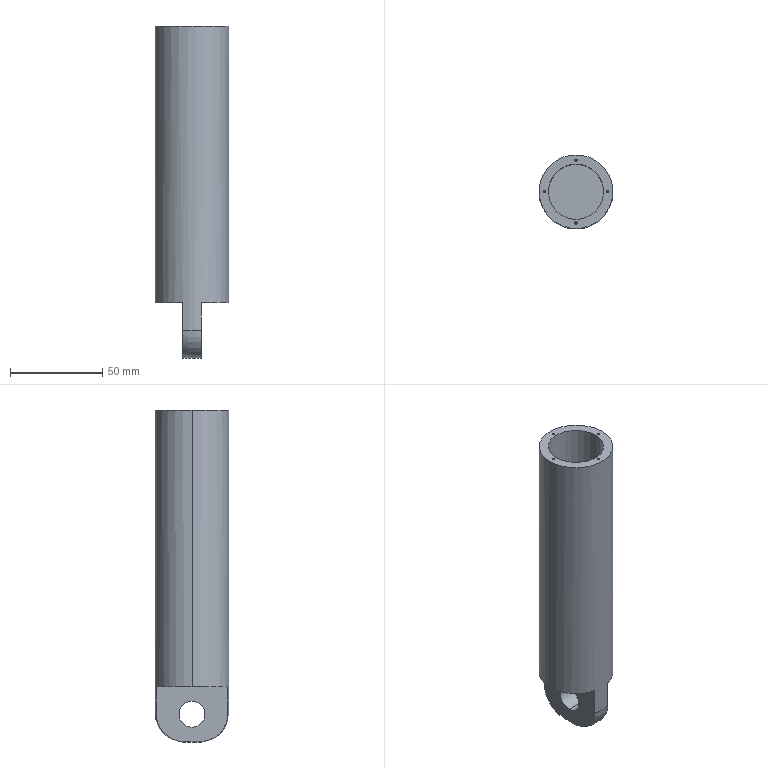Component | SolidWorks | CylinderBody-1 | 1 solid | 31 faces | box 40 x 40 x 180 mm | volume 98862 mm3 | cylinder 14 | cone 8 | plane 7 | torus 2 | commonest cylinder face diameters 1.25 x8 30 x2 14 x2 40 x2
STEP:
#1=CARTESIAN_POINT('',(0.8858,-0.06482,8.959));
#2=VERTEX_POINT('',#1);
#3=CARTESIAN_POINT('',(0.935,-0.06482,8.959));
#4=VERTEX_POINT('',#3);
#5=CARTESIAN_POINT('',(0.9104,-0.06482,8.959));
#6=DIRECTION('',(0.,0.,1.));
#7=DIRECTION('',(1.,0.,0.));
#8=AXIS2_PLACEMENT_3D('',#5,#6,#7);
#9=CIRCLE('',#8,0.02461);
#10=EDGE_CURVE('',#2,#4,#9,.T.);
#11=ORIENTED_EDGE('',*,*,#10,.F.);
#12=CARTESIAN_POINT('',(0.8858,-0.06482,9.154));
#13=VERTEX_POINT('',#12);
#14=CARTESIAN_POINT('',(0.8858,-0.06482,9.154));
#15=DIRECTION('',(0.,0.,1.));
#16=VECTOR('',#15,39.37);
#17=LINE('',#14,#16);
#18=EDGE_CURVE('',#2,#13,#17,.T.);
#19=ORIENTED_EDGE('',*,*,#18,.T.);
#20=CARTESIAN_POINT('',(0.935,-0.06482,9.154));
#21=VERTEX_POINT('',#20);
#22=CARTESIAN_POINT('',(0.9104,-0.06482,9.154));
#23=DIRECTION('',(0.,0.,1.));
#24=DIRECTION('',(1.,0.,0.));
#25=AXIS2_PLACEMENT_3D('',#22,#23,#24);
#26=CIRCLE('',#25,0.02461);
#27=EDGE_CURVE('',#13,#21,#26,.T.);
#28=ORIENTED_EDGE('',*,*,#27,.T.);
#29=CARTESIAN_POINT('',(0.935,-0.06482,9.154));
#30=DIRECTION('',(0.,0.,1.));
#31=VECTOR('',#30,39.37);
#32=LINE('',#29,#31);
#33=EDGE_CURVE('',#4,#21,#32,.T.);
#34=ORIENTED_EDGE('',*,*,#33,.F.);
#35=EDGE_LOOP('',(#11,#19,#28,#34));
#36=FACE_OUTER_BOUND('',#35,.T.);
#37=CARTESIAN_POINT('',(0.9104,-0.06482,9.154));
#38=DIRECTION('',(0.,0.,1.));
#39=DIRECTION('',(1.,0.,0.));
#40=AXIS2_PLACEMENT_3D('',#37,#38,#39);
#41=CYLINDRICAL_SURFACE('',#40,0.02461);
#42=ADVANCED_FACE('',(#36),#41,.F.);
#43=CARTESIAN_POINT('',(0.9104,-0.06482,8.944));
#44=VERTEX_POINT('',#43);
#45=CARTESIAN_POINT('',(0.935,-0.06482,8.959));
#46=DIRECTION('',(0.8572,0.,0.515));
#47=VECTOR('',#46,39.37);
#48=LINE('',#45,#47);
#49=EDGE_CURVE('',#44,#4,#48,.T.);
#50=ORIENTED_EDGE('',*,*,#49,.F.);
#51=CARTESIAN_POINT('',(0.8858,-0.06482,8.959));
#52=DIRECTION('',(-0.8572,0.,0.515));
#53=VECTOR('',#52,39.37);
#54=LINE('',#51,#53);
#55=EDGE_CURVE('',#44,#2,#54,.T.);
#56=ORIENTED_EDGE('',*,*,#55,.T.);
#57=ORIENTED_EDGE('',*,*,#10,.T.);
#58=EDGE_LOOP('',(#50,#56,#57));
#59=FACE_OUTER_BOUND('',#58,.T.);
#60=CARTESIAN_POINT('',(0.9104,-0.06482,8.959));
#61=DIRECTION('',(0.,0.,1.));
#62=DIRECTION('',(1.,0.,0.));
#63=AXIS2_PLACEMENT_3D('',#60,#61,#62);
#64=CONICAL_SURFACE('',#63,0.02461,1.03);
#65=ADVANCED_FACE('',(#59),#64,.F.);
#66=CARTESIAN_POINT('',(0.2165,-0.7341,8.959));
#67=VERTEX_POINT('',#66);
#68=CARTESIAN_POINT('',(0.2657,-0.7341,8.959));
#69=VERTEX_POINT('',#68);
#70=CARTESIAN_POINT('',(0.2411,-0.7341,8.959));
#71=DIRECTION('',(0.,0.,1.));
#72=DIRECTION('',(1.,0.,0.));
#73=AXIS2_PLACEMENT_3D('',#70,#71,#72);
#74=CIRCLE('',#73,0.02461);
#75=EDGE_CURVE('',#67,#69,#74,.T.);
#76=ORIENTED_EDGE('',*,*,#75,.F.);
#77=CARTESIAN_POINT('',(0.2165,-0.7341,9.154));
#78=VERTEX_POINT('',#77);
#79=CARTESIAN_POINT('',(0.2165,-0.7341,9.154));
#80=DIRECTION('',(0.,0.,1.));
#81=VECTOR('',#80,39.37);
#82=LINE('',#79,#81);
#83=EDGE_CURVE('',#67,#78,#82,.T.);
#84=ORIENTED_EDGE('',*,*,#83,.T.);
#85=CARTESIAN_POINT('',(0.2657,-0.7341,9.154));
#86=VERTEX_POINT('',#85);
#87=CARTESIAN_POINT('',(0.2411,-0.7341,9.154));
#88=DIRECTION('',(0.,0.,1.));
#89=DIRECTION('',(1.,0.,0.));
#90=AXIS2_PLACEMENT_3D('',#87,#88,#89);
#91=CIRCLE('',#90,0.02461);
#92=EDGE_CURVE('',#78,#86,#91,.T.);
#93=ORIENTED_EDGE('',*,*,#92,.T.);
#94=CARTESIAN_POINT('',(0.2657,-0.7341,9.154));
#95=DIRECTION('',(0.,0.,1.));
#96=VECTOR('',#95,39.37);
#97=LINE('',#94,#96);
#98=EDGE_CURVE('',#69,#86,#97,.T.);
#99=ORIENTED_EDGE('',*,*,#98,.F.);
#100=EDGE_LOOP('',(#76,#84,#93,#99));
#101=FACE_OUTER_BOUND('',#100,.T.);
#102=CARTESIAN_POINT('',(0.2411,-0.7341,9.154));
#103=DIRECTION('',(0.,0.,1.));
#104=DIRECTION('',(1.,0.,0.));
#105=AXIS2_PLACEMENT_3D('',#102,#103,#104);
#106=CYLINDRICAL_SURFACE('',#105,0.02461);
#107=ADVANCED_FACE('',(#101),#106,.F.);
#108=CARTESIAN_POINT('',(0.2411,-0.7341,8.944));
#109=VERTEX_POINT('',#108);
#110=CARTESIAN_POINT('',(0.2657,-0.7341,8.959));
#111=DIRECTION('',(0.8572,0.,0.515));
#112=VECTOR('',#111,39.37);
#113=LINE('',#110,#112);
#114=EDGE_CURVE('',#109,#69,#113,.T.);
#115=ORIENTED_EDGE('',*,*,#114,.F.);
#116=CARTESIAN_POINT('',(0.2165,-0.7341,8.959));
#117=DIRECTION('',(-0.8572,0.,0.515));
#118=VECTOR('',#117,39.37);
#119=LINE('',#116,#118);
#120=EDGE_CURVE('',#109,#67,#119,.T.);
#121=ORIENTED_EDGE('',*,*,#120,.T.);
#122=ORIENTED_EDGE('',*,*,#75,.T.);
#123=EDGE_LOOP('',(#115,#121,#122));
#124=FACE_OUTER_BOUND('',#123,.T.);
#125=CARTESIAN_POINT('',(0.2411,-0.7341,8.959));
#126=DIRECTION('',(0.,0.,1.));
#127=DIRECTION('',(1.,0.,0.));
#128=AXIS2_PLACEMENT_3D('',#125,#126,#127);
#129=CONICAL_SURFACE('',#128,0.02461,1.03);
#130=ADVANCED_FACE('',(#124),#129,.F.);
#131=CARTESIAN_POINT('',(-0.4528,-0.06482,8.959));
#132=VERTEX_POINT('',#131);
#133=CARTESIAN_POINT('',(-0.4035,-0.06482,8.959));
#134=VERTEX_POINT('',#133);
#135=CARTESIAN_POINT('',(-0.4282,-0.06482,8.959));
#136=DIRECTION('',(0.,0.,1.));
#137=DIRECTION('',(1.,0.,0.));
#138=AXIS2_PLACEMENT_3D('',#135,#136,#137);
#139=CIRCLE('',#138,0.02461);
#140=EDGE_CURVE('',#132,#134,#139,.T.);
#141=ORIENTED_EDGE('',*,*,#140,.F.);
#142=CARTESIAN_POINT('',(-0.4528,-0.06482,9.154));
#143=VERTEX_POINT('',#142);
#144=CARTESIAN_POINT('',(-0.4528,-0.06482,9.154));
#145=DIRECTION('',(0.,0.,1.));
#146=VECTOR('',#145,39.37);
#147=LINE('',#144,#146);
#148=EDGE_CURVE('',#132,#143,#147,.T.);
#149=ORIENTED_EDGE('',*,*,#148,.T.);
#150=CARTESIAN_POINT('',(-0.4035,-0.06482,9.154));
#151=VERTEX_POINT('',#150);
#152=CARTESIAN_POINT('',(-0.4282,-0.06482,9.154));
#153=DIRECTION('',(0.,0.,1.));
#154=DIRECTION('',(1.,0.,0.));
#155=AXIS2_PLACEMENT_3D('',#152,#153,#154);
#156=CIRCLE('',#155,0.02461);
#157=EDGE_CURVE('',#143,#151,#156,.T.);
#158=ORIENTED_EDGE('',*,*,#157,.T.);
#159=CARTESIAN_POINT('',(-0.4035,-0.06482,9.154));
#160=DIRECTION('',(0.,0.,1.));
#161=VECTOR('',#160,39.37);
#162=LINE('',#159,#161);
#163=EDGE_CURVE('',#134,#151,#162,.T.);
#164=ORIENTED_EDGE('',*,*,#163,.F.);
#165=EDGE_LOOP('',(#141,#149,#158,#164));
#166=FACE_OUTER_BOUND('',#165,.T.);
#167=CARTESIAN_POINT('',(-0.4282,-0.06482,9.154));
#168=DIRECTION('',(0.,0.,1.));
#169=DIRECTION('',(1.,0.,0.));
#170=AXIS2_PLACEMENT_3D('',#167,#168,#169);
#171=CYLINDRICAL_SURFACE('',#170,0.02461);
#172=ADVANCED_FACE('',(#166),#171,.F.);
#173=CARTESIAN_POINT('',(-0.4282,-0.06482,8.944));
#174=VERTEX_POINT('',#173);
#175=CARTESIAN_POINT('',(-0.4035,-0.06482,8.959));
#176=DIRECTION('',(0.8572,0.,0.515));
#177=VECTOR('',#176,39.37);
#178=LINE('',#175,#177);
#179=EDGE_CURVE('',#174,#134,#178,.T.);
#180=ORIENTED_EDGE('',*,*,#179,.F.);
#181=CARTESIAN_POINT('',(-0.4528,-0.06482,8.959));
#182=DIRECTION('',(-0.8572,0.,0.515));
#183=VECTOR('',#182,39.37);
#184=LINE('',#181,#183);
#185=EDGE_CURVE('',#174,#132,#184,.T.);
#186=ORIENTED_EDGE('',*,*,#185,.T.);
#187=ORIENTED_EDGE('',*,*,#140,.T.);
#188=EDGE_LOOP('',(#180,#186,#187));
#189=FACE_OUTER_BOUND('',#188,.T.);
#190=CARTESIAN_POINT('',(-0.4282,-0.06482,8.959));
#191=DIRECTION('',(0.,0.,1.));
#192=DIRECTION('',(1.,0.,0.));
#193=AXIS2_PLACEMENT_3D('',#190,#191,#192);
#194=CONICAL_SURFACE('',#193,0.02461,1.03);
#195=ADVANCED_FACE('',(#189),#194,.F.);
#196=CARTESIAN_POINT('',(0.2165,0.6045,8.959));
#197=VERTEX_POINT('',#196);
#198=CARTESIAN_POINT('',(0.2657,0.6045,8.959));
#199=VERTEX_POINT('',#198);
#200=CARTESIAN_POINT('',(0.2411,0.6045,8.959));
#201=DIRECTION('',(0.,0.,1.));
#202=DIRECTION('',(1.,0.,0.));
#203=AXIS2_PLACEMENT_3D('',#200,#201,#202);
#204=CIRCLE('',#203,0.02461);
#205=EDGE_CURVE('',#197,#199,#204,.T.);
#206=ORIENTED_EDGE('',*,*,#205,.F.);
#207=CARTESIAN_POINT('',(0.2165,0.6045,9.154));
#208=VERTEX_POINT('',#207);
#209=CARTESIAN_POINT('',(0.2165,0.6045,9.154));
#210=DIRECTION('',(0.,0.,1.));
#211=VECTOR('',#210,39.37);
#212=LINE('',#209,#211);
#213=EDGE_CURVE('',#197,#208,#212,.T.);
#214=ORIENTED_EDGE('',*,*,#213,.T.);
#215=CARTESIAN_POINT('',(0.2657,0.6045,9.154));
#216=VERTEX_POINT('',#215);
#217=CARTESIAN_POINT('',(0.2411,0.6045,9.154));
#218=DIRECTION('',(0.,0.,1.));
#219=DIRECTION('',(1.,0.,0.));
#220=AXIS2_PLACEMENT_3D('',#217,#218,#219);
#221=CIRCLE('',#220,0.02461);
#222=EDGE_CURVE('',#208,#216,#221,.T.);
#223=ORIENTED_EDGE('',*,*,#222,.T.);
#224=CARTESIAN_POINT('',(0.2657,0.6045,9.154));
#225=DIRECTION('',(0.,0.,1.));
#226=VECTOR('',#225,39.37);
#227=LINE('',#224,#226);
#228=EDGE_CURVE('',#199,#216,#227,.T.);
#229=ORIENTED_EDGE('',*,*,#228,.F.);
#230=EDGE_LOOP('',(#206,#214,#223,#229));
#231=FACE_OUTER_BOUND('',#230,.T.);
#232=CARTESIAN_POINT('',(0.2411,0.6045,9.154));
#233=DIRECTION('',(0.,0.,1.));
#234=DIRECTION('',(1.,0.,0.));
#235=AXIS2_PLACEMENT_3D('',#232,#233,#234);
#236=CYLINDRICAL_SURFACE('',#235,0.02461);
#237=ADVANCED_FACE('',(#231),#236,.F.);
#238=CARTESIAN_POINT('',(0.2411,0.6045,8.944));
#239=VERTEX_POINT('',#238);
#240=CARTESIAN_POINT('',(0.2657,0.6045,8.959));
#241=DIRECTION('',(0.8572,0.,0.515));
#242=VECTOR('',#241,39.37);
#243=LINE('',#240,#242);
#244=EDGE_CURVE('',#239,#199,#243,.T.);
#245=ORIENTED_EDGE('',*,*,#244,.F.);
#246=CARTESIAN_POINT('',(0.2165,0.6045,8.959));
#247=DIRECTION('',(-0.8572,0.,0.515));
#248=VECTOR('',#247,39.37);
#249=LINE('',#246,#248);
#250=EDGE_CURVE('',#239,#197,#249,.T.);
#251=ORIENTED_EDGE('',*,*,#250,.T.);
#252=ORIENTED_EDGE('',*,*,#205,.T.);
#253=EDGE_LOOP('',(#245,#251,#252));
#254=FACE_OUTER_BOUND('',#253,.T.);
#255=CARTESIAN_POINT('',(0.2411,0.6045,8.959));
#256=DIRECTION('',(0.,0.,1.));
#257=DIRECTION('',(1.,0.,0.));
#258=AXIS2_PLACEMENT_3D('',#255,#256,#257);
#259=CONICAL_SURFACE('',#258,0.02461,1.03);
#260=ADVANCED_FACE('',(#254),#259,.F.);
#261=CARTESIAN_POINT('',(-0.3494,-0.06482,3.642));
#262=VERTEX_POINT('',#261);
#263=CARTESIAN_POINT('',(0.8317,-0.06482,3.642));
#264=VERTEX_POINT('',#263);
#265=CARTESIAN_POINT('',(0.2411,-0.06482,3.642));
#266=DIRECTION('',(0.,0.,1.));
#267=DIRECTION('',(1.,0.,0.));
#268=AXIS2_PLACEMENT_3D('',#265,#266,#267);
#269=CIRCLE('',#268,0.5906);
#270=EDGE_CURVE('',#262,#264,#269,.T.);
#271=ORIENTED_EDGE('',*,*,#270,.F.);
#272=CARTESIAN_POINT('',(-0.3494,-0.06482,9.154));
#273=VERTEX_POINT('',#272);
#274=CARTESIAN_POINT('',(-0.3494,-0.06482,3.642));
#275=DIRECTION('',(0.,0.,1.));
#276=VECTOR('',#275,39.37);
#277=LINE('',#274,#276);
#278=EDGE_CURVE('',#262,#273,#277,.T.);
#279=ORIENTED_EDGE('',*,*,#278,.T.);
#280=CARTESIAN_POINT('',(0.8317,-0.06482,9.154));
#281=VERTEX_POINT('',#280);
#282=CARTESIAN_POINT('',(0.2411,-0.06482,9.154));
#283=DIRECTION('',(0.,0.,1.));
#284=DIRECTION('',(1.,0.,0.));
#285=AXIS2_PLACEMENT_3D('',#282,#283,#284);
#286=CIRCLE('',#285,0.5906);
#287=EDGE_CURVE('',#273,#281,#286,.T.);
#288=ORIENTED_EDGE('',*,*,#287,.T.);
#289=CARTESIAN_POINT('',(0.8317,-0.06482,3.642));
#290=DIRECTION('',(0.,0.,1.));
#291=VECTOR('',#290,39.37);
#292=LINE('',#289,#291);
#293=EDGE_CURVE('',#264,#281,#292,.T.);
#294=ORIENTED_EDGE('',*,*,#293,.F.);
#295=EDGE_LOOP('',(#271,#279,#288,#294));
#296=FACE_OUTER_BOUND('',#295,.T.);
#297=CARTESIAN_POINT('',(0.2411,-0.06482,3.642));
#298=DIRECTION('',(0.,0.,1.));
#299=DIRECTION('',(1.,0.,0.));
#300=AXIS2_PLACEMENT_3D('',#297,#298,#299);
#301=CYLINDRICAL_SURFACE('',#300,0.5906);
#302=ADVANCED_FACE('',(#296),#301,.F.);
#303=CARTESIAN_POINT('',(0.438,-0.06482,2.382));
#304=VERTEX_POINT('',#303);
#305=CARTESIAN_POINT('',(0.438,-0.06482,2.933));
#306=VERTEX_POINT('',#305);
#307=CARTESIAN_POINT('',(0.438,-0.06482,2.657));
#308=DIRECTION('',(-1.,0.,0.));
#309=DIRECTION('',(0.,0.,1.));
#310=AXIS2_PLACEMENT_3D('',#307,#308,#309);
#311=CIRCLE('',#310,0.2756);
#312=EDGE_CURVE('',#304,#306,#311,.T.);
#313=ORIENTED_EDGE('',*,*,#312,.F.);
#314=CARTESIAN_POINT('',(0.04429,-0.06482,2.382));
#315=VERTEX_POINT('',#314);
#316=CARTESIAN_POINT('',(1.029,-0.06482,2.382));
#317=DIRECTION('',(-1.,0.,0.));
#318=VECTOR('',#317,39.37);
#319=LINE('',#316,#318);
#320=EDGE_CURVE('',#304,#315,#319,.T.);
#321=ORIENTED_EDGE('',*,*,#320,.T.);
#322=CARTESIAN_POINT('',(0.04429,-0.06482,2.933));
#323=VERTEX_POINT('',#322);
#324=CARTESIAN_POINT('',(0.04429,-0.06482,2.657));
#325=DIRECTION('',(-1.,0.,0.));
#326=DIRECTION('',(0.,0.,1.));
#327=AXIS2_PLACEMENT_3D('',#324,#325,#326);
#328=CIRCLE('',#327,0.2756);
#329=EDGE_CURVE('',#315,#323,#328,.T.);
#330=ORIENTED_EDGE('',*,*,#329,.T.);
#331=CARTESIAN_POINT('',(1.029,-0.06482,2.933));
#332=DIRECTION('',(-1.,0.,0.));
#333=VECTOR('',#332,39.37);
#334=LINE('',#331,#333);
#335=EDGE_CURVE('',#306,#323,#334,.T.);
#336=ORIENTED_EDGE('',*,*,#335,.F.);
#337=EDGE_LOOP('',(#313,#321,#330,#336));
#338=FACE_OUTER_BOUND('',#337,.T.);
#339=CARTESIAN_POINT('',(1.029,-0.06482,2.657));
#340=DIRECTION('',(-1.,0.,0.));
#341=DIRECTION('',(0.,0.,1.));
#342=AXIS2_PLACEMENT_3D('',#339,#340,#341);
#343=CYLINDRICAL_SURFACE('',#342,0.2756);
#344=ADVANCED_FACE('',(#338),#343,.F.);
#345=CARTESIAN_POINT('',(1.029,-0.06482,9.154));
#346=VERTEX_POINT('',#345);
#347=CARTESIAN_POINT('',(-0.5463,-0.06482,9.154));
#348=VERTEX_POINT('',#347);
#349=CARTESIAN_POINT('',(0.2411,-0.06482,9.154));
#350=DIRECTION('',(0.,0.,1.));
#351=DIRECTION('',(1.,0.,0.));
#352=AXIS2_PLACEMENT_3D('',#349,#350,#351);
#353=CIRCLE('',#352,0.7874);
#354=EDGE_CURVE('',#346,#348,#353,.T.);
#355=ORIENTED_EDGE('',*,*,#354,.F.);
#356=CARTESIAN_POINT('',(1.029,-0.06482,3.248));
#357=VERTEX_POINT('',#356);
#358=CARTESIAN_POINT('',(1.029,-0.06482,9.154));
#359=DIRECTION('',(0.,0.,-1.));
#360=VECTOR('',#359,39.37);
#361=LINE('',#358,#360);
#362=EDGE_CURVE('',#346,#357,#361,.T.);
#363=ORIENTED_EDGE('',*,*,#362,.T.);
#364=CARTESIAN_POINT('',(0.438,0.6976,3.248));
#365=VERTEX_POINT('',#364);
#366=CARTESIAN_POINT('',(0.2411,-0.06482,3.248));
#367=DIRECTION('',(0.,0.,1.));
#368=DIRECTION('',(1.,0.,0.));
#369=AXIS2_PLACEMENT_3D('',#366,#367,#368);
#370=CIRCLE('',#369,0.7874);
#371=EDGE_CURVE('',#357,#365,#370,.T.);
#372=ORIENTED_EDGE('',*,*,#371,.T.);
#373=CARTESIAN_POINT('',(0.438,0.6976,2.657));
#374=VERTEX_POINT('',#373);
#375=CARTESIAN_POINT('',(0.438,0.6976,9.154));
#376=DIRECTION('',(0.,0.,-1.));
#377=VECTOR('',#376,39.37);
#378=LINE('',#375,#377);
#379=EDGE_CURVE('',#365,#374,#378,.T.);
#380=ORIENTED_EDGE('',*,*,#379,.T.);
#381=CARTESIAN_POINT('',(0.04429,0.6976,2.657));
#382=VERTEX_POINT('',#381);
#383=CARTESIAN_POINT('',(0.2411,-0.06482,2.657));
#384=DIRECTION('',(0.,0.,1.));
#385=DIRECTION('',(1.,0.,0.));
#386=AXIS2_PLACEMENT_3D('',#383,#384,#385);
#387=CIRCLE('',#386,0.7874);
#388=EDGE_CURVE('',#374,#382,#387,.T.);
#389=ORIENTED_EDGE('',*,*,#388,.T.);
#390=CARTESIAN_POINT('',(0.04429,0.6976,3.248));
#391=VERTEX_POINT('',#390);
#392=CARTESIAN_POINT('',(0.04429,0.6976,9.154));
#393=DIRECTION('',(0.,0.,1.));
#394=VECTOR('',#393,39.37);
#395=LINE('',#392,#394);
#396=EDGE_CURVE('',#382,#391,#395,.T.);
#397=ORIENTED_EDGE('',*,*,#396,.T.);
#398=CARTESIAN_POINT('',(-0.5463,-0.06482,3.248));
#399=VERTEX_POINT('',#398);
#400=CARTESIAN_POINT('',(0.2411,-0.06482,3.248));
#401=DIRECTION('',(0.,0.,1.));
#402=DIRECTION('',(1.,0.,0.));
#403=AXIS2_PLACEMENT_3D('',#400,#401,#402);
#404=CIRCLE('',#403,0.7874);
#405=EDGE_CURVE('',#391,#399,#404,.T.);
#406=ORIENTED_EDGE('',*,*,#405,.T.);
#407=CARTESIAN_POINT('',(-0.5463,-0.06482,9.154));
#408=DIRECTION('',(0.,0.,-1.));
#409=VECTOR('',#408,39.37);
#410=LINE('',#407,#409);
#411=EDGE_CURVE('',#348,#399,#410,.T.);
#412=ORIENTED_EDGE('',*,*,#411,.F.);
#413=EDGE_LOOP('',(#355,#363,#372,#380,#389,#397,#406,#412));
#414=FACE_OUTER_BOUND('',#413,.T.);
#415=CARTESIAN_POINT('',(0.2411,-0.06482,9.154));
#416=DIRECTION('',(0.,0.,-1.));
#417=DIRECTION('',(-1.,0.,0.));
#418=AXIS2_PLACEMENT_3D('',#415,#416,#417);
#419=CYLINDRICAL_SURFACE('',#418,0.7874);
#420=ADVANCED_FACE('',(#414),#419,.T.);
#421=ORIENTED_EDGE('',*,*,#362,.F.);
#422=CARTESIAN_POINT('',(0.2411,-0.06482,9.154));
#423=DIRECTION('',(0.,0.,1.));
#424=DIRECTION('',(1.,0.,0.));
#425=AXIS2_PLACEMENT_3D('',#422,#423,#424);
#426=CIRCLE('',#425,0.7874);
#427=EDGE_CURVE('',#348,#346,#426,.T.);
#428=ORIENTED_EDGE('',*,*,#427,.F.);
#429=ORIENTED_EDGE('',*,*,#411,.T.);
#430=CARTESIAN_POINT('',(0.04429,-0.8272,3.248));
#431=VERTEX_POINT('',#430);
#432=CARTESIAN_POINT('',(0.2411,-0.06482,3.248));
#433=DIRECTION('',(0.,0.,1.));
#434=DIRECTION('',(1.,0.,0.));
#435=AXIS2_PLACEMENT_3D('',#432,#433,#434);
#436=CIRCLE('',#435,0.7874);
#437=EDGE_CURVE('',#399,#431,#436,.T.);
#438=ORIENTED_EDGE('',*,*,#437,.T.);
#439=CARTESIAN_POINT('',(0.04429,-0.8272,2.657));
#440=VERTEX_POINT('',#439);
#441=CARTESIAN_POINT('',(0.04429,-0.8272,9.154));
#442=DIRECTION('',(0.,0.,-1.));
#443=VECTOR('',#442,39.37);
#444=LINE('',#441,#443);
#445=EDGE_CURVE('',#431,#440,#444,.T.);
#446=ORIENTED_EDGE('',*,*,#445,.T.);
#447=CARTESIAN_POINT('',(0.438,-0.8272,2.657));
#448=VERTEX_POINT('',#447);
#449=CARTESIAN_POINT('',(0.2411,-0.06482,2.657));
#450=DIRECTION('',(0.,0.,1.));
#451=DIRECTION('',(1.,0.,0.));
#452=AXIS2_PLACEMENT_3D('',#449,#450,#451);
#453=CIRCLE('',#452,0.7874);
#454=EDGE_CURVE('',#440,#448,#453,.T.);
#455=ORIENTED_EDGE('',*,*,#454,.T.);
#456=CARTESIAN_POINT('',(0.438,-0.8272,3.248));
#457=VERTEX_POINT('',#456);
#458=CARTESIAN_POINT('',(0.438,-0.8272,9.154));
#459=DIRECTION('',(0.,0.,1.));
#460=VECTOR('',#459,39.37);
#461=LINE('',#458,#460);
#462=EDGE_CURVE('',#448,#457,#461,.T.);
#463=ORIENTED_EDGE('',*,*,#462,.T.);
#464=CARTESIAN_POINT('',(0.2411,-0.06482,3.248));
#465=DIRECTION('',(0.,0.,1.));
#466=DIRECTION('',(1.,0.,0.));
#467=AXIS2_PLACEMENT_3D('',#464,#465,#466);
#468=CIRCLE('',#467,0.7874);
#469=EDGE_CURVE('',#457,#357,#468,.T.);
#470=ORIENTED_EDGE('',*,*,#469,.T.);
#471=EDGE_LOOP('',(#421,#428,#429,#438,#446,#455,#463,#470));
#472=FACE_OUTER_BOUND('',#471,.T.);
#473=CARTESIAN_POINT('',(0.2411,-0.06482,9.154));
#474=DIRECTION('',(0.,0.,-1.));
#475=DIRECTION('',(-1.,0.,0.));
#476=AXIS2_PLACEMENT_3D('',#473,#474,#475);
#477=CYLINDRICAL_SURFACE('',#476,0.7874);
#478=ADVANCED_FACE('',(#472),#477,.T.);
#479=CARTESIAN_POINT('',(0.9104,-0.06482,9.154));
#480=DIRECTION('',(0.,0.,1.));
#481=DIRECTION('',(1.,0.,0.));
#482=AXIS2_PLACEMENT_3D('',#479,#480,#481);
#483=CIRCLE('',#482,0.02461);
#484=EDGE_CURVE('',#21,#13,#483,.T.);
#485=ORIENTED_EDGE('',*,*,#484,.F.);
#486=ORIENTED_EDGE('',*,*,#27,.F.);
#487=EDGE_LOOP('',(#485,#486));
#488=FACE_BOUND('',#487,.T.);
#489=CARTESIAN_POINT('',(0.2411,-0.7341,9.154));
#490=DIRECTION('',(0.,0.,1.));
#491=DIRECTION('',(1.,0.,0.));
#492=AXIS2_PLACEMENT_3D('',#489,#490,#491);
#493=CIRCLE('',#492,0.02461);
#494=EDGE_CURVE('',#86,#78,#493,.T.);
#495=ORIENTED_EDGE('',*,*,#494,.F.);
#496=ORIENTED_EDGE('',*,*,#92,.F.);
#497=EDGE_LOOP('',(#495,#496));
#498=FACE_BOUND('',#497,.T.);
#499=CARTESIAN_POINT('',(-0.4282,-0.06482,9.154));
#500=DIRECTION('',(0.,0.,1.));
#501=DIRECTION('',(1.,0.,0.));
#502=AXIS2_PLACEMENT_3D('',#499,#500,#501);
#503=CIRCLE('',#502,0.02461);
#504=EDGE_CURVE('',#151,#143,#503,.T.);
#505=ORIENTED_EDGE('',*,*,#504,.F.);
#506=ORIENTED_EDGE('',*,*,#157,.F.);
#507=EDGE_LOOP('',(#505,#506));
#508=FACE_BOUND('',#507,.T.);
#509=CARTESIAN_POINT('',(0.2411,0.6045,9.154));
#510=DIRECTION('',(0.,0.,1.));
#511=DIRECTION('',(1.,0.,0.));
#512=AXIS2_PLACEMENT_3D('',#509,#510,#511);
#513=CIRCLE('',#512,0.02461);
#514=EDGE_CURVE('',#216,#208,#513,.T.);
#515=ORIENTED_EDGE('',*,*,#514,.F.);
#516=ORIENTED_EDGE('',*,*,#222,.F.);
#517=EDGE_LOOP('',(#515,#516));
#518=FACE_BOUND('',#517,.T.);
#519=CARTESIAN_POINT('',(0.2411,-0.06482,9.154));
#520=DIRECTION('',(0.,0.,1.));
#521=DIRECTION('',(1.,0.,0.));
#522=AXIS2_PLACEMENT_3D('',#519,#520,#521);
#523=CIRCLE('',#522,0.5906);
#524=EDGE_CURVE('',#281,#273,#523,.T.);
#525=ORIENTED_EDGE('',*,*,#524,.F.);
#526=ORIENTED_EDGE('',*,*,#287,.F.);
#527=EDGE_LOOP('',(#525,#526));
#528=FACE_BOUND('',#527,.T.);
#529=ORIENTED_EDGE('',*,*,#427,.T.);
#530=ORIENTED_EDGE('',*,*,#354,.T.);
#531=EDGE_LOOP('',(#529,#530));
#532=FACE_OUTER_BOUND('',#531,.T.);
#533=CARTESIAN_POINT('',(0.2411,-0.06482,9.154));
#534=DIRECTION('',(0.,0.,1.));
#535=DIRECTION('',(1.,0.,0.));
#536=AXIS2_PLACEMENT_3D('',#533,#534,#535);
#537=PLANE('',#536);
#538=ADVANCED_FACE('',(#488,#498,#508,#518,#528,#532),#537,.T.);
#539=CARTESIAN_POINT('',(0.438,-0.06482,2.067));
#540=VERTEX_POINT('',#539);
#541=CARTESIAN_POINT('',(0.04429,-0.06482,2.067));
#542=VERTEX_POINT('',#541);
#543=CARTESIAN_POINT('',(0.2411,-0.06482,2.067));
#544=DIRECTION('',(0.,0.,-1.));
#545=DIRECTION('',(1.,0.,0.));
#546=AXIS2_PLACEMENT_3D('',#543,#544,#545);
#547=CIRCLE('',#546,0.1969);
#548=EDGE_CURVE('',#540,#542,#547,.T.);
#549=ORIENTED_EDGE('',*,*,#548,.T.);
#550=CARTESIAN_POINT('',(0.2411,-0.06482,2.067));
#551=DIRECTION('',(0.,0.,-1.));
#552=DIRECTION('',(1.,0.,0.));
#553=AXIS2_PLACEMENT_3D('',#550,#551,#552);
#554=CIRCLE('',#553,0.1969);
#555=EDGE_CURVE('',#542,#540,#554,.T.);
#556=ORIENTED_EDGE('',*,*,#555,.T.);
#557=EDGE_LOOP('',(#549,#556));
#558=FACE_OUTER_BOUND('',#557,.T.);
#559=CARTESIAN_POINT('',(0.2411,-0.06482,2.067));
#560=DIRECTION('',(0.,0.,1.));
#561=DIRECTION('',(1.,0.,0.));
#562=AXIS2_PLACEMENT_3D('',#559,#560,#561);
#563=PLANE('',#562);
#564=ADVANCED_FACE('',(#558),#563,.F.);
#565=CARTESIAN_POINT('',(0.04429,-0.8522,3.248));
#566=DIRECTION('',(0.,1.,0.));
#567=VECTOR('',#566,39.37);
#568=LINE('',#565,#567);
#569=EDGE_CURVE('',#431,#391,#568,.T.);
#570=ORIENTED_EDGE('',*,*,#569,.F.);
#571=ORIENTED_EDGE('',*,*,#437,.F.);
#572=ORIENTED_EDGE('',*,*,#405,.F.);
#573=EDGE_LOOP('',(#570,#571,#572));
#574=FACE_OUTER_BOUND('',#573,.T.);
#575=CARTESIAN_POINT('',(-0.5463,-0.8522,3.248));
#576=DIRECTION('',(0.,0.,1.));
#577=DIRECTION('',(1.,0.,0.));
#578=AXIS2_PLACEMENT_3D('',#575,#576,#577);
#579=PLANE('',#578);
#580=ADVANCED_FACE('',(#574),#579,.F.);
#581=CARTESIAN_POINT('',(0.04429,-0.06482,2.657));
#582=DIRECTION('',(-1.,0.,0.));
#583=DIRECTION('',(0.,0.,1.));
#584=AXIS2_PLACEMENT_3D('',#581,#582,#583);
#585=CIRCLE('',#584,0.2756);
#586=EDGE_CURVE('',#323,#315,#585,.T.);
#587=ORIENTED_EDGE('',*,*,#586,.F.);
#588=ORIENTED_EDGE('',*,*,#329,.F.);
#589=EDGE_LOOP('',(#587,#588));
#590=FACE_BOUND('',#589,.T.);
#591=ORIENTED_EDGE('',*,*,#396,.F.);
#592=CARTESIAN_POINT('',(0.04429,0.6976,2.657));
#593=CARTESIAN_POINT('',(0.04429,0.6976,2.611));
#594=CARTESIAN_POINT('',(0.04429,0.6921,2.566));
#595=CARTESIAN_POINT('',(0.04429,0.6787,2.511));
#596=CARTESIAN_POINT('',(0.04429,0.6756,2.5));
#597=CARTESIAN_POINT('',(0.04429,0.6689,2.478));
#598=CARTESIAN_POINT('',(0.04429,0.6652,2.467));
#599=CARTESIAN_POINT('',(0.04429,0.6532,2.435));
#600=CARTESIAN_POINT('',(0.04429,0.6439,2.414));
#601=CARTESIAN_POINT('',(0.04429,0.6231,2.374));
#602=CARTESIAN_POINT('',(0.04429,0.6115,2.355));
#603=CARTESIAN_POINT('',(0.04429,0.5859,2.317));
#604=CARTESIAN_POINT('',(0.04429,0.5719,2.299));
#605=CARTESIAN_POINT('',(0.04429,0.5269,2.247));
#606=CARTESIAN_POINT('',(0.04429,0.4934,2.216));
#607=CARTESIAN_POINT('',(0.04429,0.4379,2.176));
#608=CARTESIAN_POINT('',(0.04429,0.4184,2.164));
#609=CARTESIAN_POINT('',(0.04429,0.3786,2.142));
#610=CARTESIAN_POINT('',(0.04429,0.3581,2.132));
#611=CARTESIAN_POINT('',(0.04429,0.3163,2.114));
#612=CARTESIAN_POINT('',(0.04429,0.2949,2.106));
#613=CARTESIAN_POINT('',(0.04429,0.2511,2.093));
#614=CARTESIAN_POINT('',(0.04429,0.2288,2.088));
#615=CARTESIAN_POINT('',(0.04429,0.1617,2.075));
#616=CARTESIAN_POINT('',(0.04429,0.1166,2.07));
#617=CARTESIAN_POINT('',(0.04429,0.0487,2.068));
#618=CARTESIAN_POINT('',(0.04429,0.02601,2.067));
#619=CARTESIAN_POINT('',(0.04429,-0.01939,2.067));
#620=CARTESIAN_POINT('',(0.04429,-0.04211,2.067));
#621=CARTESIAN_POINT('',(0.04429,-0.06482,2.067));
#622=B_SPLINE_CURVE_WITH_KNOTS('',3,(#592,#593,#594,#595,#596,#597,#598,#599,#600,#601,#602,#603,#604,#605,#606,#607,#608,#609,#610,#611,#612,#613,#614,#615,#616,#617,#618,#619,#620,#621),.UNSPECIFIED.,.F.,.F.,(4,2,2,2,2,2,2,2,2,2,2,2,2,2,4),(0.,0.003456,0.004319,0.005183,0.006911,0.008639,0.01037,0.01382,0.01555,0.01728,0.01901,0.02073,0.02419,0.02592,0.02764),.UNSPECIFIED.);
#623=EDGE_CURVE('',#382,#542,#622,.T.);
#624=ORIENTED_EDGE('',*,*,#623,.T.);
#625=CARTESIAN_POINT('',(0.04429,-0.06482,2.067));
#626=CARTESIAN_POINT('',(0.04429,-0.08766,2.067));
#627=CARTESIAN_POINT('',(0.04429,-0.1105,2.067));
#628=CARTESIAN_POINT('',(0.04429,-0.1562,2.067));
#629=CARTESIAN_POINT('',(0.04429,-0.179,2.068));
#630=CARTESIAN_POINT('',(0.04429,-0.2246,2.069));
#631=CARTESIAN_POINT('',(0.04429,-0.2474,2.071));
#632=CARTESIAN_POINT('',(0.04429,-0.2929,2.076));
#633=CARTESIAN_POINT('',(0.04429,-0.3154,2.079));
#634=CARTESIAN_POINT('',(0.04429,-0.3599,2.088));
#635=CARTESIAN_POINT('',(0.04429,-0.3819,2.093));
#636=CARTESIAN_POINT('',(0.04429,-0.4254,2.107));
#637=CARTESIAN_POINT('',(0.04429,-0.447,2.114));
#638=CARTESIAN_POINT('',(0.04429,-0.5101,2.141));
#639=CARTESIAN_POINT('',(0.04429,-0.5496,2.163));
#640=CARTESIAN_POINT('',(0.04429,-0.5956,2.196));
#641=CARTESIAN_POINT('',(0.04429,-0.6046,2.203));
#642=CARTESIAN_POINT('',(0.04429,-0.6224,2.218));
#643=CARTESIAN_POINT('',(0.04429,-0.6311,2.225));
#644=CARTESIAN_POINT('',(0.04429,-0.6563,2.248));
#645=CARTESIAN_POINT('',(0.04429,-0.6721,2.265));
#646=CARTESIAN_POINT('',(0.04429,-0.7017,2.299));
#647=CARTESIAN_POINT('',(0.04429,-0.7155,2.317));
#648=CARTESIAN_POINT('',(0.04429,-0.7346,2.345));
#649=CARTESIAN_POINT('',(0.04429,-0.7407,2.355));
#650=CARTESIAN_POINT('',(0.04429,-0.7524,2.374));
#651=CARTESIAN_POINT('',(0.04429,-0.758,2.384));
#652=CARTESIAN_POINT('',(0.04429,-0.7842,2.435));
#653=CARTESIAN_POINT('',(0.04429,-0.8,2.477));
#654=CARTESIAN_POINT('',(0.04429,-0.8162,2.544));
#655=CARTESIAN_POINT('',(0.04429,-0.8204,2.566));
#656=CARTESIAN_POINT('',(0.04429,-0.8258,2.612));
#657=CARTESIAN_POINT('',(0.04429,-0.8272,2.635));
#658=CARTESIAN_POINT('',(0.04429,-0.8272,2.657));
#659=B_SPLINE_CURVE_WITH_KNOTS('',3,(#625,#626,#627,#628,#629,#630,#631,#632,#633,#634,#635,#636,#637,#638,#639,#640,#641,#642,#643,#644,#645,#646,#647,#648,#649,#650,#651,#652,#653,#654,#655,#656,#657,#658),.UNSPECIFIED.,.F.,.F.,(4,2,2,2,2,2,2,2,2,2,2,2,2,2,2,2,4),(0.,0.001739,0.003479,0.005218,0.006957,0.008696,0.01044,0.01391,0.01478,0.01565,0.01739,0.01913,0.02,0.02087,0.02435,0.02609,0.02783),.UNSPECIFIED.);
#660=EDGE_CURVE('',#542,#440,#659,.T.);
#661=ORIENTED_EDGE('',*,*,#660,.T.);
#662=ORIENTED_EDGE('',*,*,#445,.F.);
#663=ORIENTED_EDGE('',*,*,#569,.T.);
#664=EDGE_LOOP('',(#591,#624,#661,#662,#663));
#665=FACE_OUTER_BOUND('',#664,.T.);
#666=CARTESIAN_POINT('',(0.04429,-0.8522,2.067));
#667=DIRECTION('',(1.,0.,-0.));
#668=DIRECTION('',(-0.,0.,-1.));
#669=AXIS2_PLACEMENT_3D('',#666,#667,#668);
#670=PLANE('',#669);
#671=ADVANCED_FACE('',(#590,#665),#670,.F.);
#672=ORIENTED_EDGE('',*,*,#469,.F.);
#673=CARTESIAN_POINT('',(0.438,-0.8522,3.248));
#674=DIRECTION('',(0.,1.,0.));
#675=VECTOR('',#674,39.37);
#676=LINE('',#673,#675);
#677=EDGE_CURVE('',#457,#365,#676,.T.);
#678=ORIENTED_EDGE('',*,*,#677,.T.);
#679=ORIENTED_EDGE('',*,*,#371,.F.);
#680=EDGE_LOOP('',(#672,#678,#679));
#681=FACE_OUTER_BOUND('',#680,.T.);
#682=CARTESIAN_POINT('',(1.029,-0.8522,3.248));
#683=DIRECTION('',(0.,0.,1.));
#684=DIRECTION('',(1.,0.,-0.));
#685=AXIS2_PLACEMENT_3D('',#682,#683,#684);
#686=PLANE('',#685);
#687=ADVANCED_FACE('',(#681),#686,.F.);
#688=CARTESIAN_POINT('',(0.438,-0.06482,2.657));
#689=DIRECTION('',(-1.,0.,0.));
#690=DIRECTION('',(0.,0.,1.));
#691=AXIS2_PLACEMENT_3D('',#688,#689,#690);
#692=CIRCLE('',#691,0.2756);
#693=EDGE_CURVE('',#306,#304,#692,.T.);
#694=ORIENTED_EDGE('',*,*,#693,.T.);
#695=ORIENTED_EDGE('',*,*,#312,.T.);
#696=EDGE_LOOP('',(#694,#695));
#697=FACE_BOUND('',#696,.T.);
#698=CARTESIAN_POINT('',(0.438,-0.8272,2.657));
#699=CARTESIAN_POINT('',(0.438,-0.8272,2.611));
#700=CARTESIAN_POINT('',(0.438,-0.8217,2.566));
#701=CARTESIAN_POINT('',(0.438,-0.8083,2.511));
#702=CARTESIAN_POINT('',(0.438,-0.8053,2.5));
#703=CARTESIAN_POINT('',(0.438,-0.7986,2.478));
#704=CARTESIAN_POINT('',(0.438,-0.7949,2.467));
#705=CARTESIAN_POINT('',(0.438,-0.7828,2.435));
#706=CARTESIAN_POINT('',(0.438,-0.7735,2.414));
#707=CARTESIAN_POINT('',(0.438,-0.7527,2.374));
#708=CARTESIAN_POINT('',(0.438,-0.7411,2.355));
#709=CARTESIAN_POINT('',(0.438,-0.7156,2.317));
#710=CARTESIAN_POINT('',(0.438,-0.7015,2.299));
#711=CARTESIAN_POINT('',(0.438,-0.6566,2.247));
#712=CARTESIAN_POINT('',(0.438,-0.6231,2.216));
#713=CARTESIAN_POINT('',(0.438,-0.5675,2.176));
#714=CARTESIAN_POINT('',(0.438,-0.548,2.164));
#715=CARTESIAN_POINT('',(0.438,-0.5082,2.142));
#716=CARTESIAN_POINT('',(0.438,-0.4878,2.132));
#717=CARTESIAN_POINT('',(0.438,-0.4459,2.114));
#718=CARTESIAN_POINT('',(0.438,-0.4245,2.106));
#719=CARTESIAN_POINT('',(0.438,-0.3808,2.093));
#720=CARTESIAN_POINT('',(0.438,-0.3584,2.088));
#721=CARTESIAN_POINT('',(0.438,-0.2913,2.075));
#722=CARTESIAN_POINT('',(0.438,-0.2463,2.07));
#723=CARTESIAN_POINT('',(0.438,-0.1783,2.068));
#724=CARTESIAN_POINT('',(0.438,-0.1557,2.067));
#725=CARTESIAN_POINT('',(0.438,-0.1103,2.067));
#726=CARTESIAN_POINT('',(0.438,-0.08754,2.067));
#727=CARTESIAN_POINT('',(0.438,-0.06482,2.067));
#728=B_SPLINE_CURVE_WITH_KNOTS('',3,(#698,#699,#700,#701,#702,#703,#704,#705,#706,#707,#708,#709,#710,#711,#712,#713,#714,#715,#716,#717,#718,#719,#720,#721,#722,#723,#724,#725,#726,#727),.UNSPECIFIED.,.F.,.F.,(4,2,2,2,2,2,2,2,2,2,2,2,2,2,4),(0.,0.003456,0.004319,0.005183,0.006911,0.008639,0.01037,0.01382,0.01555,0.01728,0.01901,0.02073,0.02419,0.02592,0.02764),.UNSPECIFIED.);
#729=EDGE_CURVE('',#448,#540,#728,.T.);
#730=ORIENTED_EDGE('',*,*,#729,.T.);
#731=CARTESIAN_POINT('',(0.438,-0.06482,2.067));
#732=CARTESIAN_POINT('',(0.438,-0.04199,2.067));
#733=CARTESIAN_POINT('',(0.438,-0.01915,2.067));
#734=CARTESIAN_POINT('',(0.438,0.02651,2.067));
#735=CARTESIAN_POINT('',(0.438,0.04933,2.068));
#736=CARTESIAN_POINT('',(0.438,0.09495,2.069));
#737=CARTESIAN_POINT('',(0.438,0.1178,2.071));
#738=CARTESIAN_POINT('',(0.438,0.1632,2.076));
#739=CARTESIAN_POINT('',(0.438,0.1857,2.079));
#740=CARTESIAN_POINT('',(0.438,0.2303,2.088));
#741=CARTESIAN_POINT('',(0.438,0.2523,2.093));
#742=CARTESIAN_POINT('',(0.438,0.2958,2.107));
#743=CARTESIAN_POINT('',(0.438,0.3174,2.114));
#744=CARTESIAN_POINT('',(0.438,0.3805,2.141));
#745=CARTESIAN_POINT('',(0.438,0.42,2.163));
#746=CARTESIAN_POINT('',(0.438,0.466,2.196));
#747=CARTESIAN_POINT('',(0.438,0.475,2.203));
#748=CARTESIAN_POINT('',(0.438,0.4927,2.218));
#749=CARTESIAN_POINT('',(0.438,0.5014,2.225));
#750=CARTESIAN_POINT('',(0.438,0.5267,2.248));
#751=CARTESIAN_POINT('',(0.438,0.5425,2.265));
#752=CARTESIAN_POINT('',(0.438,0.5721,2.299));
#753=CARTESIAN_POINT('',(0.438,0.5858,2.317));
#754=CARTESIAN_POINT('',(0.438,0.6049,2.345));
#755=CARTESIAN_POINT('',(0.438,0.611,2.355));
#756=CARTESIAN_POINT('',(0.438,0.6227,2.374));
#757=CARTESIAN_POINT('',(0.438,0.6283,2.384));
#758=CARTESIAN_POINT('',(0.438,0.6545,2.435));
#759=CARTESIAN_POINT('',(0.438,0.6704,2.477));
#760=CARTESIAN_POINT('',(0.438,0.6866,2.544));
#761=CARTESIAN_POINT('',(0.438,0.6907,2.566));
#762=CARTESIAN_POINT('',(0.438,0.6962,2.612));
#763=CARTESIAN_POINT('',(0.438,0.6976,2.635));
#764=CARTESIAN_POINT('',(0.438,0.6976,2.657));
#765=B_SPLINE_CURVE_WITH_KNOTS('',3,(#731,#732,#733,#734,#735,#736,#737,#738,#739,#740,#741,#742,#743,#744,#745,#746,#747,#748,#749,#750,#751,#752,#753,#754,#755,#756,#757,#758,#759,#760,#761,#762,#763,#764),.UNSPECIFIED.,.F.,.F.,(4,2,2,2,2,2,2,2,2,2,2,2,2,2,2,2,4),(0.,0.001739,0.003479,0.005218,0.006957,0.008696,0.01044,0.01391,0.01478,0.01565,0.01739,0.01913,0.02,0.02087,0.02435,0.02609,0.02783),.UNSPECIFIED.);
#766=EDGE_CURVE('',#540,#374,#765,.T.);
#767=ORIENTED_EDGE('',*,*,#766,.T.);
#768=ORIENTED_EDGE('',*,*,#379,.F.);
#769=ORIENTED_EDGE('',*,*,#677,.F.);
#770=ORIENTED_EDGE('',*,*,#462,.F.);
#771=EDGE_LOOP('',(#730,#767,#768,#769,#770));
#772=FACE_OUTER_BOUND('',#771,.T.);
#773=CARTESIAN_POINT('',(0.438,-0.8522,2.067));
#774=DIRECTION('',(-1.,0.,0.));
#775=DIRECTION('',(0.,0.,1.));
#776=AXIS2_PLACEMENT_3D('',#773,#774,#775);
#777=PLANE('',#776);
#778=ADVANCED_FACE('',(#697,#772),#777,.F.);
#779=ORIENTED_EDGE('',*,*,#766,.F.);
#780=ORIENTED_EDGE('',*,*,#555,.F.);
#781=ORIENTED_EDGE('',*,*,#623,.F.);
#782=ORIENTED_EDGE('',*,*,#388,.F.);
#783=EDGE_LOOP('',(#779,#780,#781,#782));
#784=FACE_OUTER_BOUND('',#783,.T.);
#785=CARTESIAN_POINT('',(0.2411,-0.06482,2.657));
#786=DIRECTION('',(0.,0.,1.));
#787=DIRECTION('',(1.,0.,0.));
#788=AXIS2_PLACEMENT_3D('',#785,#786,#787);
#789=TOROIDAL_SURFACE('',#788,0.1969,0.5906);
#790=ADVANCED_FACE('',(#784),#789,.T.);
#791=ORIENTED_EDGE('',*,*,#660,.F.);
#792=ORIENTED_EDGE('',*,*,#548,.F.);
#793=ORIENTED_EDGE('',*,*,#729,.F.);
#794=ORIENTED_EDGE('',*,*,#454,.F.);
#795=EDGE_LOOP('',(#791,#792,#793,#794));
#796=FACE_OUTER_BOUND('',#795,.T.);
#797=CARTESIAN_POINT('',(0.2411,-0.06482,2.657));
#798=DIRECTION('',(0.,0.,1.));
#799=DIRECTION('',(1.,0.,0.));
#800=AXIS2_PLACEMENT_3D('',#797,#798,#799);
#801=TOROIDAL_SURFACE('',#800,0.1969,0.5906);
#802=ADVANCED_FACE('',(#796),#801,.T.);
#803=ORIENTED_EDGE('',*,*,#320,.F.);
#804=ORIENTED_EDGE('',*,*,#693,.F.);
#805=ORIENTED_EDGE('',*,*,#335,.T.);
#806=ORIENTED_EDGE('',*,*,#586,.T.);
#807=EDGE_LOOP('',(#803,#804,#805,#806));
#808=FACE_OUTER_BOUND('',#807,.T.);
#809=CARTESIAN_POINT('',(1.029,-0.06482,2.657));
#810=DIRECTION('',(-1.,0.,0.));
#811=DIRECTION('',(0.,0.,1.));
#812=AXIS2_PLACEMENT_3D('',#809,#810,#811);
#813=CYLINDRICAL_SURFACE('',#812,0.2756);
#814=ADVANCED_FACE('',(#808),#813,.F.);
#815=ORIENTED_EDGE('',*,*,#278,.F.);
#816=CARTESIAN_POINT('',(0.2411,-0.06482,3.642));
#817=DIRECTION('',(0.,0.,1.));
#818=DIRECTION('',(1.,0.,0.));
#819=AXIS2_PLACEMENT_3D('',#816,#817,#818);
#820=CIRCLE('',#819,0.5906);
#821=EDGE_CURVE('',#264,#262,#820,.T.);
#822=ORIENTED_EDGE('',*,*,#821,.F.);
#823=ORIENTED_EDGE('',*,*,#293,.T.);
#824=ORIENTED_EDGE('',*,*,#524,.T.);
#825=EDGE_LOOP('',(#815,#822,#823,#824));
#826=FACE_OUTER_BOUND('',#825,.T.);
#827=CARTESIAN_POINT('',(0.2411,-0.06482,3.642));
#828=DIRECTION('',(0.,0.,1.));
#829=DIRECTION('',(1.,0.,0.));
#830=AXIS2_PLACEMENT_3D('',#827,#828,#829);
#831=CYLINDRICAL_SURFACE('',#830,0.5906);
#832=ADVANCED_FACE('',(#826),#831,.F.);
#833=ORIENTED_EDGE('',*,*,#821,.T.);
#834=ORIENTED_EDGE('',*,*,#270,.T.);
#835=EDGE_LOOP('',(#833,#834));
#836=FACE_OUTER_BOUND('',#835,.T.);
#837=CARTESIAN_POINT('',(0.2411,-0.06482,3.642));
#838=DIRECTION('',(0.,0.,1.));
#839=DIRECTION('',(1.,0.,0.));
#840=AXIS2_PLACEMENT_3D('',#837,#838,#839);
#841=PLANE('',#840);
#842=ADVANCED_FACE('',(#836),#841,.T.);
#843=ORIENTED_EDGE('',*,*,#250,.F.);
#844=ORIENTED_EDGE('',*,*,#244,.T.);
#845=CARTESIAN_POINT('',(0.2411,0.6045,8.959));
#846=DIRECTION('',(0.,0.,1.));
#847=DIRECTION('',(1.,0.,0.));
#848=AXIS2_PLACEMENT_3D('',#845,#846,#847);
#849=CIRCLE('',#848,0.02461);
#850=EDGE_CURVE('',#199,#197,#849,.T.);
#851=ORIENTED_EDGE('',*,*,#850,.T.);
#852=EDGE_LOOP('',(#843,#844,#851));
#853=FACE_OUTER_BOUND('',#852,.T.);
#854=CARTESIAN_POINT('',(0.2411,0.6045,8.959));
#855=DIRECTION('',(0.,0.,1.));
#856=DIRECTION('',(1.,0.,0.));
#857=AXIS2_PLACEMENT_3D('',#854,#855,#856);
#858=CONICAL_SURFACE('',#857,0.02461,1.03);
#859=ADVANCED_FACE('',(#853),#858,.F.);
#860=ORIENTED_EDGE('',*,*,#213,.F.);
#861=ORIENTED_EDGE('',*,*,#850,.F.);
#862=ORIENTED_EDGE('',*,*,#228,.T.);
#863=ORIENTED_EDGE('',*,*,#514,.T.);
#864=EDGE_LOOP('',(#860,#861,#862,#863));
#865=FACE_OUTER_BOUND('',#864,.T.);
#866=CARTESIAN_POINT('',(0.2411,0.6045,9.154));
#867=DIRECTION('',(0.,0.,1.));
#868=DIRECTION('',(1.,0.,0.));
#869=AXIS2_PLACEMENT_3D('',#866,#867,#868);
#870=CYLINDRICAL_SURFACE('',#869,0.02461);
#871=ADVANCED_FACE('',(#865),#870,.F.);
#872=ORIENTED_EDGE('',*,*,#185,.F.);
#873=ORIENTED_EDGE('',*,*,#179,.T.);
#874=CARTESIAN_POINT('',(-0.4282,-0.06482,8.959));
#875=DIRECTION('',(0.,0.,1.));
#876=DIRECTION('',(1.,0.,0.));
#877=AXIS2_PLACEMENT_3D('',#874,#875,#876);
#878=CIRCLE('',#877,0.02461);
#879=EDGE_CURVE('',#134,#132,#878,.T.);
#880=ORIENTED_EDGE('',*,*,#879,.T.);
#881=EDGE_LOOP('',(#872,#873,#880));
#882=FACE_OUTER_BOUND('',#881,.T.);
#883=CARTESIAN_POINT('',(-0.4282,-0.06482,8.959));
#884=DIRECTION('',(0.,0.,1.));
#885=DIRECTION('',(1.,0.,0.));
#886=AXIS2_PLACEMENT_3D('',#883,#884,#885);
#887=CONICAL_SURFACE('',#886,0.02461,1.03);
#888=ADVANCED_FACE('',(#882),#887,.F.);
#889=ORIENTED_EDGE('',*,*,#148,.F.);
#890=ORIENTED_EDGE('',*,*,#879,.F.);
#891=ORIENTED_EDGE('',*,*,#163,.T.);
#892=ORIENTED_EDGE('',*,*,#504,.T.);
#893=EDGE_LOOP('',(#889,#890,#891,#892));
#894=FACE_OUTER_BOUND('',#893,.T.);
#895=CARTESIAN_POINT('',(-0.4282,-0.06482,9.154));
#896=DIRECTION('',(0.,0.,1.));
#897=DIRECTION('',(1.,0.,0.));
#898=AXIS2_PLACEMENT_3D('',#895,#896,#897);
#899=CYLINDRICAL_SURFACE('',#898,0.02461);
#900=ADVANCED_FACE('',(#894),#899,.F.);
#901=ORIENTED_EDGE('',*,*,#120,.F.);
#902=ORIENTED_EDGE('',*,*,#114,.T.);
#903=CARTESIAN_POINT('',(0.2411,-0.7341,8.959));
#904=DIRECTION('',(0.,0.,1.));
#905=DIRECTION('',(1.,0.,0.));
#906=AXIS2_PLACEMENT_3D('',#903,#904,#905);
#907=CIRCLE('',#906,0.02461);
#908=EDGE_CURVE('',#69,#67,#907,.T.);
#909=ORIENTED_EDGE('',*,*,#908,.T.);
#910=EDGE_LOOP('',(#901,#902,#909));
#911=FACE_OUTER_BOUND('',#910,.T.);
#912=CARTESIAN_POINT('',(0.2411,-0.7341,8.959));
#913=DIRECTION('',(0.,0.,1.));
#914=DIRECTION('',(1.,0.,0.));
#915=AXIS2_PLACEMENT_3D('',#912,#913,#914);
#916=CONICAL_SURFACE('',#915,0.02461,1.03);
#917=ADVANCED_FACE('',(#911),#916,.F.);
#918=ORIENTED_EDGE('',*,*,#83,.F.);
#919=ORIENTED_EDGE('',*,*,#908,.F.);
#920=ORIENTED_EDGE('',*,*,#98,.T.);
#921=ORIENTED_EDGE('',*,*,#494,.T.);
#922=EDGE_LOOP('',(#918,#919,#920,#921));
#923=FACE_OUTER_BOUND('',#922,.T.);
#924=CARTESIAN_POINT('',(0.2411,-0.7341,9.154));
#925=DIRECTION('',(0.,0.,1.));
#926=DIRECTION('',(1.,0.,0.));
#927=AXIS2_PLACEMENT_3D('',#924,#925,#926);
#928=CYLINDRICAL_SURFACE('',#927,0.02461);
#929=ADVANCED_FACE('',(#923),#928,.F.);
#930=ORIENTED_EDGE('',*,*,#55,.F.);
#931=ORIENTED_EDGE('',*,*,#49,.T.);
#932=CARTESIAN_POINT('',(0.9104,-0.06482,8.959));
#933=DIRECTION('',(0.,0.,1.));
#934=DIRECTION('',(1.,0.,0.));
#935=AXIS2_PLACEMENT_3D('',#932,#933,#934);
#936=CIRCLE('',#935,0.02461);
#937=EDGE_CURVE('',#4,#2,#936,.T.);
#938=ORIENTED_EDGE('',*,*,#937,.T.);
#939=EDGE_LOOP('',(#930,#931,#938));
#940=FACE_OUTER_BOUND('',#939,.T.);
#941=CARTESIAN_POINT('',(0.9104,-0.06482,8.959));
#942=DIRECTION('',(0.,0.,1.));
#943=DIRECTION('',(1.,0.,0.));
#944=AXIS2_PLACEMENT_3D('',#941,#942,#943);
#945=CONICAL_SURFACE('',#944,0.02461,1.03);
#946=ADVANCED_FACE('',(#940),#945,.F.);
#947=ORIENTED_EDGE('',*,*,#18,.F.);
#948=ORIENTED_EDGE('',*,*,#937,.F.);
#949=ORIENTED_EDGE('',*,*,#33,.T.);
#950=ORIENTED_EDGE('',*,*,#484,.T.);
#951=EDGE_LOOP('',(#947,#948,#949,#950));
#952=FACE_OUTER_BOUND('',#951,.T.);
#953=CARTESIAN_POINT('',(0.9104,-0.06482,9.154));
#954=DIRECTION('',(0.,0.,1.));
#955=DIRECTION('',(1.,0.,0.));
#956=AXIS2_PLACEMENT_3D('',#953,#954,#955);
#957=CYLINDRICAL_SURFACE('',#956,0.02461);
#958=ADVANCED_FACE('',(#952),#957,.F.);
#959=CLOSED_SHELL('',(#42,#65,#107,#130,#172,#195,#237,#260,#302,#344,#420,#478,#538,#564,#580,#671,#687,#778,#790,#802,#814,#832,#842,#859,#871,#888,#900,#917,#929,#946,#958));
#960=MANIFOLD_SOLID_BREP('',#959);
#961=CARTESIAN_POINT('',(0.,0.,0.));
#962=DIRECTION('',(0.,0.,1.));
#963=DIRECTION('',(1.,0.,0.));
#964=AXIS2_PLACEMENT_3D('',#961,#962,#963);
#965=(LENGTH_UNIT()NAMED_UNIT(*)SI_UNIT($,.METRE.));
#966=LENGTH_MEASURE_WITH_UNIT(LENGTH_MEASURE(0.0254),#965);
#967=DIMENSIONAL_EXPONENTS(1.,0.,0.,0.,0.,0.,0.);
#968=(CONVERSION_BASED_UNIT('',#966)LENGTH_UNIT()NAMED_UNIT(#967));
#969=UNCERTAINTY_MEASURE_WITH_UNIT(LENGTH_MEASURE(0.00001),#968,'','');
#970=(NAMED_UNIT(*)PLANE_ANGLE_UNIT()SI_UNIT($,.RADIAN.));
#971=(NAMED_UNIT(*)SI_UNIT($,.STERADIAN.)SOLID_ANGLE_UNIT());
#972=(GEOMETRIC_REPRESENTATION_CONTEXT(3)GLOBAL_UNCERTAINTY_ASSIGNED_CONTEXT((#969))GLOBAL_UNIT_ASSIGNED_CONTEXT((#968,#970,#971))REPRESENTATION_CONTEXT('',''));
#973=ADVANCED_BREP_SHAPE_REPRESENTATION('',(#960,#964),#972);
#974=COLOUR_RGB('',0.7922,0.8196,0.9333);
#975=FILL_AREA_STYLE_COLOUR('',#974);
#976=FILL_AREA_STYLE('',(#975));
#977=SURFACE_STYLE_FILL_AREA(#976);
#978=SURFACE_SIDE_STYLE('',(#977));
#979=SURFACE_STYLE_USAGE(.BOTH.,#978);
#980=PRESENTATION_STYLE_ASSIGNMENT((#979));
#981=STYLED_ITEM('',(#980),#960);
#982=(LENGTH_UNIT()NAMED_UNIT(*)SI_UNIT($,.METRE.));
#983=LENGTH_MEASURE_WITH_UNIT(LENGTH_MEASURE(0.0254),#982);
#984=DIMENSIONAL_EXPONENTS(1.,0.,0.,0.,0.,0.,0.);
#985=(CONVERSION_BASED_UNIT('',#983)LENGTH_UNIT()NAMED_UNIT(#984));
#986=UNCERTAINTY_MEASURE_WITH_UNIT(LENGTH_MEASURE(0.00001),#985,'','');
#987=(NAMED_UNIT(*)PLANE_ANGLE_UNIT()SI_UNIT($,.RADIAN.));
#988=(NAMED_UNIT(*)SI_UNIT($,.STERADIAN.)SOLID_ANGLE_UNIT());
#989=(GEOMETRIC_REPRESENTATION_CONTEXT(3)GLOBAL_UNCERTAINTY_ASSIGNED_CONTEXT((#986))GLOBAL_UNIT_ASSIGNED_CONTEXT((#985,#987,#988))REPRESENTATION_CONTEXT('',''));
#990=MECHANICAL_DESIGN_GEOMETRIC_PRESENTATION_REPRESENTATION('',(#981),#989);
#991=PRESENTATION_LAYER_ASSIGNMENT('','',(#981));